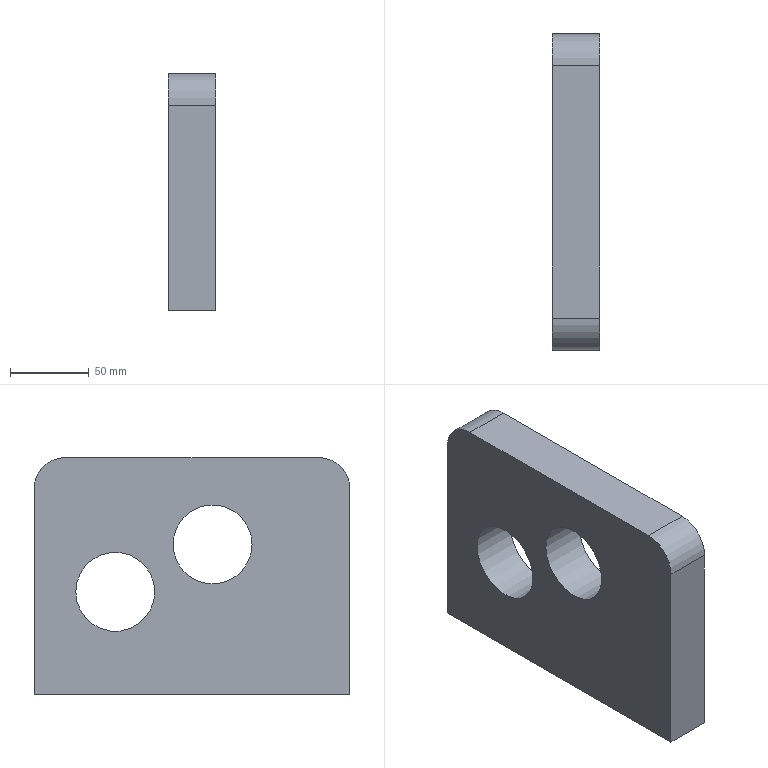Component | NX | TEMPLATE | 1 solid | 16 faces | box 30 x 200 x 150 mm | volume 766710 mm3 | plane 6 | cylinder 6 | cone 4 | commonest cylinder face diameters 50 x2 14 x2 40 x2
STEP:
#1=CARTESIAN_POINT('',(0.,0.,0.));
#2=DIRECTION('',(0.,0.,1.));
#3=DIRECTION('',(1.,0.,0.));
#4=AXIS2_PLACEMENT_3D('',#1,#2,#3);
#5=CARTESIAN_POINT('',(-275.,-100.,180.));
#6=VERTEX_POINT('',#5);
#7=CARTESIAN_POINT('',(-275.,-100.,50.));
#8=VERTEX_POINT('',#7);
#9=CARTESIAN_POINT('',(-275.,-100.,200.));
#10=DIRECTION('',(0.,-0.,-1.));
#11=VECTOR('',#10,1.);
#12=LINE('',#9,#11);
#13=CARTESIAN_POINT('',(-275.,-100.,200.));
#14=DIRECTION('',(0.,1.,-0.));
#15=DIRECTION('',(0.,-0.,-1.));
#16=AXIS2_PLACEMENT_3D('',#13,#14,#15);
#17=PLANE('',#16);
#18=CARTESIAN_POINT('',(0.,0.));
#19=DIRECTION('',(1.,0.));
#20=VECTOR('',#19,1.);
#21=LINE('',#18,#20);
#22=(GEOMETRIC_REPRESENTATION_CONTEXT(2)PARAMETRIC_REPRESENTATION_CONTEXT()REPRESENTATION_CONTEXT('',''));
#23=DEFINITIONAL_REPRESENTATION('',(#21),#22);
#24=PCURVE('',#17,#23);
#25=CARTESIAN_POINT('',(-275.,48.56,115.));
#26=DIRECTION('',(-1.,0.,0.));
#27=DIRECTION('',(0.,0.,1.));
#28=AXIS2_PLACEMENT_3D('',#25,#26,#27);
#29=PLANE('',#28);
#30=CARTESIAN_POINT('',(85.,-148.56));
#31=DIRECTION('',(-1.,-0.));
#32=VECTOR('',#31,1.);
#33=LINE('',#30,#32);
#34=(GEOMETRIC_REPRESENTATION_CONTEXT(2)PARAMETRIC_REPRESENTATION_CONTEXT()REPRESENTATION_CONTEXT('',''));
#35=DEFINITIONAL_REPRESENTATION('',(#33),#34);
#36=PCURVE('',#29,#35);
#37=SURFACE_CURVE('',#12,(#24,#36),.PCURVE_S1.);
#38=EDGE_CURVE('',#6,#8,#37,.T.);
#39=ORIENTED_EDGE('',*,*,#38,.F.);
#40=CARTESIAN_POINT('',(-305.,-100.,180.));
#41=VERTEX_POINT('',#40);
#42=CARTESIAN_POINT('',(-275.,-100.,180.));
#43=DIRECTION('',(-1.,0.,0.));
#44=VECTOR('',#43,1.);
#45=LINE('',#42,#44);
#46=CARTESIAN_POINT('',(20.,0.));
#47=DIRECTION('',(0.,1.));
#48=VECTOR('',#47,1.);
#49=LINE('',#46,#48);
#50=(GEOMETRIC_REPRESENTATION_CONTEXT(2)PARAMETRIC_REPRESENTATION_CONTEXT()REPRESENTATION_CONTEXT('',''));
#51=DEFINITIONAL_REPRESENTATION('',(#49),#50);
#52=PCURVE('',#17,#51);
#53=CARTESIAN_POINT('',(-275.,-80.,180.));
#54=DIRECTION('',(-1.,0.,0.));
#55=DIRECTION('',(0.,0.,1.));
#56=AXIS2_PLACEMENT_3D('',#53,#54,#55);
#57=CYLINDRICAL_SURFACE('',#56,20.);
#58=CARTESIAN_POINT('',(4.712,0.));
#59=DIRECTION('',(0.,1.));
#60=VECTOR('',#59,1.);
#61=LINE('',#58,#60);
#62=(GEOMETRIC_REPRESENTATION_CONTEXT(2)PARAMETRIC_REPRESENTATION_CONTEXT()REPRESENTATION_CONTEXT('',''));
#63=DEFINITIONAL_REPRESENTATION('',(#61),#62);
#64=PCURVE('',#57,#63);
#65=SURFACE_CURVE('',#45,(#52,#64),.PCURVE_S1.);
#66=EDGE_CURVE('',#6,#41,#65,.T.);
#67=ORIENTED_EDGE('',*,*,#66,.T.);
#68=CARTESIAN_POINT('',(-305.,-100.,50.));
#69=VERTEX_POINT('',#68);
#70=CARTESIAN_POINT('',(-305.,-100.,200.));
#71=DIRECTION('',(0.,-0.,-1.));
#72=VECTOR('',#71,1.);
#73=LINE('',#70,#72);
#74=CARTESIAN_POINT('',(0.,30.));
#75=DIRECTION('',(1.,0.));
#76=VECTOR('',#75,1.);
#77=LINE('',#74,#76);
#78=(GEOMETRIC_REPRESENTATION_CONTEXT(2)PARAMETRIC_REPRESENTATION_CONTEXT()REPRESENTATION_CONTEXT('',''));
#79=DEFINITIONAL_REPRESENTATION('',(#77),#78);
#80=PCURVE('',#17,#79);
#81=CARTESIAN_POINT('',(-305.,48.56,115.));
#82=DIRECTION('',(-1.,0.,0.));
#83=DIRECTION('',(0.,0.,1.));
#84=AXIS2_PLACEMENT_3D('',#81,#82,#83);
#85=PLANE('',#84);
#86=CARTESIAN_POINT('',(85.,-148.56));
#87=DIRECTION('',(-1.,-0.));
#88=VECTOR('',#87,1.);
#89=LINE('',#86,#88);
#90=(GEOMETRIC_REPRESENTATION_CONTEXT(2)PARAMETRIC_REPRESENTATION_CONTEXT()REPRESENTATION_CONTEXT('',''));
#91=DEFINITIONAL_REPRESENTATION('',(#89),#90);
#92=PCURVE('',#85,#91);
#93=SURFACE_CURVE('',#73,(#80,#92),.PCURVE_S1.);
#94=EDGE_CURVE('',#41,#69,#93,.T.);
#95=ORIENTED_EDGE('',*,*,#94,.T.);
#96=CARTESIAN_POINT('',(-275.,-100.,50.));
#97=DIRECTION('',(-1.,0.,0.));
#98=VECTOR('',#97,1.);
#99=LINE('',#96,#98);
#100=CARTESIAN_POINT('',(150.,0.));
#101=DIRECTION('',(0.,1.));
#102=VECTOR('',#101,1.);
#103=LINE('',#100,#102);
#104=(GEOMETRIC_REPRESENTATION_CONTEXT(2)PARAMETRIC_REPRESENTATION_CONTEXT()REPRESENTATION_CONTEXT('',''));
#105=DEFINITIONAL_REPRESENTATION('',(#103),#104);
#106=PCURVE('',#17,#105);
#107=CARTESIAN_POINT('',(-275.,-100.,50.));
#108=DIRECTION('',(0.,0.,1.));
#109=DIRECTION('',(1.,0.,0.));
#110=AXIS2_PLACEMENT_3D('',#107,#108,#109);
#111=PLANE('',#110);
#112=CARTESIAN_POINT('',(0.,0.));
#113=DIRECTION('',(-1.,0.));
#114=VECTOR('',#113,1.);
#115=LINE('',#112,#114);
#116=(GEOMETRIC_REPRESENTATION_CONTEXT(2)PARAMETRIC_REPRESENTATION_CONTEXT()REPRESENTATION_CONTEXT('',''));
#117=DEFINITIONAL_REPRESENTATION('',(#115),#116);
#118=PCURVE('',#111,#117);
#119=SURFACE_CURVE('',#99,(#106,#118),.PCURVE_S1.);
#120=EDGE_CURVE('',#8,#69,#119,.T.);
#121=ORIENTED_EDGE('',*,*,#120,.F.);
#122=EDGE_LOOP('',(#39,#67,#95,#121));
#123=FACE_BOUND('',#122,.T.);
#124=ADVANCED_FACE('',(#123),#17,.F.);
#125=CARTESIAN_POINT('',(-282.,50.,50.));
#126=VERTEX_POINT('',#125);
#127=CARTESIAN_POINT('',(-290.,50.,50.));
#128=DIRECTION('',(0.,0.,1.));
#129=DIRECTION('',(1.,0.,0.));
#130=AXIS2_PLACEMENT_3D('',#127,#128,#129);
#131=CIRCLE('',#130,8.);
#132=CARTESIAN_POINT('',(-15.,150.));
#133=DIRECTION('',(1.,0.));
#134=AXIS2_PLACEMENT_2D('',#132,#133);
#135=CIRCLE('',#134,8.);
#136=(GEOMETRIC_REPRESENTATION_CONTEXT(2)PARAMETRIC_REPRESENTATION_CONTEXT()REPRESENTATION_CONTEXT('',''));
#137=DEFINITIONAL_REPRESENTATION('',(#135),#136);
#138=PCURVE('',#111,#137);
#139=CARTESIAN_POINT('',(-290.,50.,50.));
#140=DIRECTION('',(0.,0.,-1.));
#141=DIRECTION('',(-1.,0.,0.));
#142=AXIS2_PLACEMENT_3D('',#139,#140,#141);
#143=CONICAL_SURFACE('',#142,8.,0.7854);
#144=CARTESIAN_POINT('',(9.425,0.));
#145=DIRECTION('',(-1.,0.));
#146=VECTOR('',#145,1.);
#147=LINE('',#144,#146);
#148=(GEOMETRIC_REPRESENTATION_CONTEXT(2)PARAMETRIC_REPRESENTATION_CONTEXT()REPRESENTATION_CONTEXT('',''));
#149=DEFINITIONAL_REPRESENTATION('',(#147),#148);
#150=PCURVE('',#143,#149);
#151=SURFACE_CURVE('',#131,(#138,#150),.PCURVE_S1.);
#152=EDGE_CURVE('',#126,#126,#151,.T.);
#153=ORIENTED_EDGE('',*,*,#152,.T.);
#154=EDGE_LOOP('',(#153));
#155=FACE_BOUND('',#154,.T.);
#156=CARTESIAN_POINT('',(-282.,-50.,50.));
#157=VERTEX_POINT('',#156);
#158=CARTESIAN_POINT('',(-290.,-50.,50.));
#159=DIRECTION('',(0.,0.,1.));
#160=DIRECTION('',(1.,0.,0.));
#161=AXIS2_PLACEMENT_3D('',#158,#159,#160);
#162=CIRCLE('',#161,8.);
#163=CARTESIAN_POINT('',(-15.,50.));
#164=DIRECTION('',(1.,0.));
#165=AXIS2_PLACEMENT_2D('',#163,#164);
#166=CIRCLE('',#165,8.);
#167=(GEOMETRIC_REPRESENTATION_CONTEXT(2)PARAMETRIC_REPRESENTATION_CONTEXT()REPRESENTATION_CONTEXT('',''));
#168=DEFINITIONAL_REPRESENTATION('',(#166),#167);
#169=PCURVE('',#111,#168);
#170=CARTESIAN_POINT('',(-290.,-50.,50.));
#171=DIRECTION('',(0.,0.,-1.));
#172=DIRECTION('',(-1.,0.,0.));
#173=AXIS2_PLACEMENT_3D('',#170,#171,#172);
#174=CONICAL_SURFACE('',#173,8.,0.7854);
#175=CARTESIAN_POINT('',(9.425,0.));
#176=DIRECTION('',(-1.,0.));
#177=VECTOR('',#176,1.);
#178=LINE('',#175,#177);
#179=(GEOMETRIC_REPRESENTATION_CONTEXT(2)PARAMETRIC_REPRESENTATION_CONTEXT()REPRESENTATION_CONTEXT('',''));
#180=DEFINITIONAL_REPRESENTATION('',(#178),#179);
#181=PCURVE('',#174,#180);
#182=SURFACE_CURVE('',#162,(#169,#181),.PCURVE_S1.);
#183=EDGE_CURVE('',#157,#157,#182,.T.);
#184=ORIENTED_EDGE('',*,*,#183,.T.);
#185=EDGE_LOOP('',(#184));
#186=FACE_BOUND('',#185,.T.);
#187=CARTESIAN_POINT('',(-305.,100.,50.));
#188=VERTEX_POINT('',#187);
#189=CARTESIAN_POINT('',(-305.,-100.,50.));
#190=DIRECTION('',(0.,1.,0.));
#191=VECTOR('',#190,1.);
#192=LINE('',#189,#191);
#193=CARTESIAN_POINT('',(-30.,0.));
#194=DIRECTION('',(0.,1.));
#195=VECTOR('',#194,1.);
#196=LINE('',#193,#195);
#197=(GEOMETRIC_REPRESENTATION_CONTEXT(2)PARAMETRIC_REPRESENTATION_CONTEXT()REPRESENTATION_CONTEXT('',''));
#198=DEFINITIONAL_REPRESENTATION('',(#196),#197);
#199=PCURVE('',#111,#198);
#200=CARTESIAN_POINT('',(-65.,-148.56));
#201=DIRECTION('',(0.,1.));
#202=VECTOR('',#201,1.);
#203=LINE('',#200,#202);
#204=(GEOMETRIC_REPRESENTATION_CONTEXT(2)PARAMETRIC_REPRESENTATION_CONTEXT()REPRESENTATION_CONTEXT('',''));
#205=DEFINITIONAL_REPRESENTATION('',(#203),#204);
#206=PCURVE('',#85,#205);
#207=SURFACE_CURVE('',#192,(#199,#206),.PCURVE_S1.);
#208=EDGE_CURVE('',#69,#188,#207,.T.);
#209=ORIENTED_EDGE('',*,*,#208,.T.);
#210=CARTESIAN_POINT('',(-275.,100.,50.));
#211=VERTEX_POINT('',#210);
#212=CARTESIAN_POINT('',(-275.,100.,50.));
#213=DIRECTION('',(-1.,0.,0.));
#214=VECTOR('',#213,1.);
#215=LINE('',#212,#214);
#216=CARTESIAN_POINT('',(0.,200.));
#217=DIRECTION('',(-1.,0.));
#218=VECTOR('',#217,1.);
#219=LINE('',#216,#218);
#220=(GEOMETRIC_REPRESENTATION_CONTEXT(2)PARAMETRIC_REPRESENTATION_CONTEXT()REPRESENTATION_CONTEXT('',''));
#221=DEFINITIONAL_REPRESENTATION('',(#219),#220);
#222=PCURVE('',#111,#221);
#223=CARTESIAN_POINT('',(-275.,100.,50.));
#224=DIRECTION('',(0.,-1.,-0.));
#225=DIRECTION('',(0.,-0.,1.));
#226=AXIS2_PLACEMENT_3D('',#223,#224,#225);
#227=PLANE('',#226);
#228=CARTESIAN_POINT('',(0.,0.));
#229=DIRECTION('',(0.,1.));
#230=VECTOR('',#229,1.);
#231=LINE('',#228,#230);
#232=(GEOMETRIC_REPRESENTATION_CONTEXT(2)PARAMETRIC_REPRESENTATION_CONTEXT()REPRESENTATION_CONTEXT('',''));
#233=DEFINITIONAL_REPRESENTATION('',(#231),#232);
#234=PCURVE('',#227,#233);
#235=SURFACE_CURVE('',#215,(#222,#234),.PCURVE_S1.);
#236=EDGE_CURVE('',#211,#188,#235,.T.);
#237=ORIENTED_EDGE('',*,*,#236,.F.);
#238=CARTESIAN_POINT('',(-275.,-100.,50.));
#239=DIRECTION('',(0.,1.,0.));
#240=VECTOR('',#239,1.);
#241=LINE('',#238,#240);
#242=CARTESIAN_POINT('',(0.,0.));
#243=DIRECTION('',(0.,1.));
#244=VECTOR('',#243,1.);
#245=LINE('',#242,#244);
#246=(GEOMETRIC_REPRESENTATION_CONTEXT(2)PARAMETRIC_REPRESENTATION_CONTEXT()REPRESENTATION_CONTEXT('',''));
#247=DEFINITIONAL_REPRESENTATION('',(#245),#246);
#248=PCURVE('',#111,#247);
#249=CARTESIAN_POINT('',(-65.,-148.56));
#250=DIRECTION('',(0.,1.));
#251=VECTOR('',#250,1.);
#252=LINE('',#249,#251);
#253=(GEOMETRIC_REPRESENTATION_CONTEXT(2)PARAMETRIC_REPRESENTATION_CONTEXT()REPRESENTATION_CONTEXT('',''));
#254=DEFINITIONAL_REPRESENTATION('',(#252),#253);
#255=PCURVE('',#29,#254);
#256=SURFACE_CURVE('',#241,(#248,#255),.PCURVE_S1.);
#257=EDGE_CURVE('',#8,#211,#256,.T.);
#258=ORIENTED_EDGE('',*,*,#257,.F.);
#259=ORIENTED_EDGE('',*,*,#120,.T.);
#260=EDGE_LOOP('',(#209,#237,#258,#259));
#261=FACE_BOUND('',#260,.T.);
#262=ADVANCED_FACE('',(#155,#186,#261),#111,.F.);
#263=CARTESIAN_POINT('',(-305.,100.,180.));
#264=VERTEX_POINT('',#263);
#265=CARTESIAN_POINT('',(-305.,100.,50.));
#266=DIRECTION('',(0.,-0.,1.));
#267=VECTOR('',#266,1.);
#268=LINE('',#265,#267);
#269=CARTESIAN_POINT('',(0.,30.));
#270=DIRECTION('',(1.,0.));
#271=VECTOR('',#270,1.);
#272=LINE('',#269,#271);
#273=(GEOMETRIC_REPRESENTATION_CONTEXT(2)PARAMETRIC_REPRESENTATION_CONTEXT()REPRESENTATION_CONTEXT('',''));
#274=DEFINITIONAL_REPRESENTATION('',(#272),#273);
#275=PCURVE('',#227,#274);
#276=CARTESIAN_POINT('',(-65.,51.44));
#277=DIRECTION('',(1.,-0.));
#278=VECTOR('',#277,1.);
#279=LINE('',#276,#278);
#280=(GEOMETRIC_REPRESENTATION_CONTEXT(2)PARAMETRIC_REPRESENTATION_CONTEXT()REPRESENTATION_CONTEXT('',''));
#281=DEFINITIONAL_REPRESENTATION('',(#279),#280);
#282=PCURVE('',#85,#281);
#283=SURFACE_CURVE('',#268,(#275,#282),.PCURVE_S1.);
#284=EDGE_CURVE('',#188,#264,#283,.T.);
#285=ORIENTED_EDGE('',*,*,#284,.T.);
#286=CARTESIAN_POINT('',(-275.,100.,180.));
#287=VERTEX_POINT('',#286);
#288=CARTESIAN_POINT('',(-275.,100.,180.));
#289=DIRECTION('',(1.,0.,0.));
#290=VECTOR('',#289,1.);
#291=LINE('',#288,#290);
#292=CARTESIAN_POINT('',(130.,0.));
#293=DIRECTION('',(0.,-1.));
#294=VECTOR('',#293,1.);
#295=LINE('',#292,#294);
#296=(GEOMETRIC_REPRESENTATION_CONTEXT(2)PARAMETRIC_REPRESENTATION_CONTEXT()REPRESENTATION_CONTEXT('',''));
#297=DEFINITIONAL_REPRESENTATION('',(#295),#296);
#298=PCURVE('',#227,#297);
#299=CARTESIAN_POINT('',(-275.,80.,180.));
#300=DIRECTION('',(-1.,0.,0.));
#301=DIRECTION('',(0.,0.,1.));
#302=AXIS2_PLACEMENT_3D('',#299,#300,#301);
#303=CYLINDRICAL_SURFACE('',#302,20.);
#304=CARTESIAN_POINT('',(1.571,0.));
#305=DIRECTION('',(0.,-1.));
#306=VECTOR('',#305,1.);
#307=LINE('',#304,#306);
#308=(GEOMETRIC_REPRESENTATION_CONTEXT(2)PARAMETRIC_REPRESENTATION_CONTEXT()REPRESENTATION_CONTEXT('',''));
#309=DEFINITIONAL_REPRESENTATION('',(#307),#308);
#310=PCURVE('',#303,#309);
#311=SURFACE_CURVE('',#291,(#298,#310),.PCURVE_S1.);
#312=EDGE_CURVE('',#264,#287,#311,.T.);
#313=ORIENTED_EDGE('',*,*,#312,.T.);
#314=CARTESIAN_POINT('',(-275.,100.,50.));
#315=DIRECTION('',(0.,-0.,1.));
#316=VECTOR('',#315,1.);
#317=LINE('',#314,#316);
#318=CARTESIAN_POINT('',(0.,0.));
#319=DIRECTION('',(1.,0.));
#320=VECTOR('',#319,1.);
#321=LINE('',#318,#320);
#322=(GEOMETRIC_REPRESENTATION_CONTEXT(2)PARAMETRIC_REPRESENTATION_CONTEXT()REPRESENTATION_CONTEXT('',''));
#323=DEFINITIONAL_REPRESENTATION('',(#321),#322);
#324=PCURVE('',#227,#323);
#325=CARTESIAN_POINT('',(-65.,51.44));
#326=DIRECTION('',(1.,-0.));
#327=VECTOR('',#326,1.);
#328=LINE('',#325,#327);
#329=(GEOMETRIC_REPRESENTATION_CONTEXT(2)PARAMETRIC_REPRESENTATION_CONTEXT()REPRESENTATION_CONTEXT('',''));
#330=DEFINITIONAL_REPRESENTATION('',(#328),#329);
#331=PCURVE('',#29,#330);
#332=SURFACE_CURVE('',#317,(#324,#331),.PCURVE_S1.);
#333=EDGE_CURVE('',#211,#287,#332,.T.);
#334=ORIENTED_EDGE('',*,*,#333,.F.);
#335=ORIENTED_EDGE('',*,*,#236,.T.);
#336=EDGE_LOOP('',(#285,#313,#334,#335));
#337=FACE_BOUND('',#336,.T.);
#338=ADVANCED_FACE('',(#337),#227,.F.);
#339=CARTESIAN_POINT('',(-275.,73.56,115.));
#340=VERTEX_POINT('',#339);
#341=CARTESIAN_POINT('',(-275.,48.56,115.));
#342=DIRECTION('',(-1.,0.,0.));
#343=DIRECTION('',(0.,1.,0.));
#344=AXIS2_PLACEMENT_3D('',#341,#342,#343);
#345=CIRCLE('',#344,25.);
#346=CARTESIAN_POINT('',(-275.,48.56,115.));
#347=DIRECTION('',(-1.,0.,0.));
#348=DIRECTION('',(0.,0.,1.));
#349=AXIS2_PLACEMENT_3D('',#346,#347,#348);
#350=CYLINDRICAL_SURFACE('',#349,25.);
#351=CARTESIAN_POINT('',(1.571,0.));
#352=DIRECTION('',(1.,0.));
#353=VECTOR('',#352,1.);
#354=LINE('',#351,#353);
#355=(GEOMETRIC_REPRESENTATION_CONTEXT(2)PARAMETRIC_REPRESENTATION_CONTEXT()REPRESENTATION_CONTEXT('',''));
#356=DEFINITIONAL_REPRESENTATION('',(#354),#355);
#357=PCURVE('',#350,#356);
#358=CARTESIAN_POINT('',(0.,0.));
#359=DIRECTION('',(0.,1.));
#360=AXIS2_PLACEMENT_2D('',#358,#359);
#361=CIRCLE('',#360,25.);
#362=(GEOMETRIC_REPRESENTATION_CONTEXT(2)PARAMETRIC_REPRESENTATION_CONTEXT()REPRESENTATION_CONTEXT('',''));
#363=DEFINITIONAL_REPRESENTATION('',(#361),#362);
#364=PCURVE('',#29,#363);
#365=SURFACE_CURVE('',#345,(#357,#364),.PCURVE_S1.);
#366=EDGE_CURVE('',#340,#340,#365,.T.);
#367=ORIENTED_EDGE('',*,*,#366,.T.);
#368=CARTESIAN_POINT('',(-305.,73.56,115.));
#369=VERTEX_POINT('',#368);
#370=CARTESIAN_POINT('',(-275.,73.56,115.));
#371=CARTESIAN_POINT('',(-305.,73.56,115.));
#372=B_SPLINE_CURVE_WITH_KNOTS('',1,(#370,#371),.UNSPECIFIED.,.F.,.F.,(2,2),(0.,30.),.PIECEWISE_BEZIER_KNOTS.);
#373=CARTESIAN_POINT('',(7.854,0.));
#374=DIRECTION('',(0.,1.));
#375=VECTOR('',#374,1.);
#376=LINE('',#373,#375);
#377=(GEOMETRIC_REPRESENTATION_CONTEXT(2)PARAMETRIC_REPRESENTATION_CONTEXT()REPRESENTATION_CONTEXT('',''));
#378=DEFINITIONAL_REPRESENTATION('',(#376),#377);
#379=PCURVE('',#350,#378);
#380=CARTESIAN_POINT('',(1.571,0.));
#381=DIRECTION('',(0.,1.));
#382=VECTOR('',#381,1.);
#383=LINE('',#380,#382);
#384=(GEOMETRIC_REPRESENTATION_CONTEXT(2)PARAMETRIC_REPRESENTATION_CONTEXT()REPRESENTATION_CONTEXT('',''));
#385=DEFINITIONAL_REPRESENTATION('',(#383),#384);
#386=PCURVE('',#350,#385);
#387=SEAM_CURVE('',#372,(#379,#386),.PCURVE_S1.);
#388=EDGE_CURVE('',#340,#369,#387,.T.);
#389=ORIENTED_EDGE('',*,*,#388,.T.);
#390=CARTESIAN_POINT('',(-305.,48.56,115.));
#391=DIRECTION('',(-1.,0.,0.));
#392=DIRECTION('',(0.,1.,0.));
#393=AXIS2_PLACEMENT_3D('',#390,#391,#392);
#394=CIRCLE('',#393,25.);
#395=CARTESIAN_POINT('',(1.571,30.));
#396=DIRECTION('',(1.,0.));
#397=VECTOR('',#396,1.);
#398=LINE('',#395,#397);
#399=(GEOMETRIC_REPRESENTATION_CONTEXT(2)PARAMETRIC_REPRESENTATION_CONTEXT()REPRESENTATION_CONTEXT('',''));
#400=DEFINITIONAL_REPRESENTATION('',(#398),#399);
#401=PCURVE('',#350,#400);
#402=CARTESIAN_POINT('',(0.,0.));
#403=DIRECTION('',(0.,1.));
#404=AXIS2_PLACEMENT_2D('',#402,#403);
#405=CIRCLE('',#404,25.);
#406=(GEOMETRIC_REPRESENTATION_CONTEXT(2)PARAMETRIC_REPRESENTATION_CONTEXT()REPRESENTATION_CONTEXT('',''));
#407=DEFINITIONAL_REPRESENTATION('',(#405),#406);
#408=PCURVE('',#85,#407);
#409=SURFACE_CURVE('',#394,(#401,#408),.PCURVE_S1.);
#410=EDGE_CURVE('',#369,#369,#409,.T.);
#411=ORIENTED_EDGE('',*,*,#410,.F.);
#412=ORIENTED_EDGE('',*,*,#388,.F.);
#413=EDGE_LOOP('',(#367,#389,#411,#412));
#414=FACE_BOUND('',#413,.F.);
#415=ADVANCED_FACE('',(#414),#350,.F.);
#416=CARTESIAN_POINT('',(-275.,80.,200.));
#417=VERTEX_POINT('',#416);
#418=CARTESIAN_POINT('',(-275.,-80.,200.));
#419=VERTEX_POINT('',#418);
#420=CARTESIAN_POINT('',(-275.,100.,200.));
#421=DIRECTION('',(0.,-1.,-0.));
#422=VECTOR('',#421,1.);
#423=LINE('',#420,#422);
#424=CARTESIAN_POINT('',(-275.,100.,200.));
#425=DIRECTION('',(0.,0.,-1.));
#426=DIRECTION('',(0.,-1.,-0.));
#427=AXIS2_PLACEMENT_3D('',#424,#425,#426);
#428=PLANE('',#427);
#429=CARTESIAN_POINT('',(0.,0.));
#430=DIRECTION('',(1.,0.));
#431=VECTOR('',#430,1.);
#432=LINE('',#429,#431);
#433=(GEOMETRIC_REPRESENTATION_CONTEXT(2)PARAMETRIC_REPRESENTATION_CONTEXT()REPRESENTATION_CONTEXT('',''));
#434=DEFINITIONAL_REPRESENTATION('',(#432),#433);
#435=PCURVE('',#428,#434);
#436=CARTESIAN_POINT('',(85.,51.44));
#437=DIRECTION('',(-0.,-1.));
#438=VECTOR('',#437,1.);
#439=LINE('',#436,#438);
#440=(GEOMETRIC_REPRESENTATION_CONTEXT(2)PARAMETRIC_REPRESENTATION_CONTEXT()REPRESENTATION_CONTEXT('',''));
#441=DEFINITIONAL_REPRESENTATION('',(#439),#440);
#442=PCURVE('',#29,#441);
#443=SURFACE_CURVE('',#423,(#435,#442),.PCURVE_S1.);
#444=EDGE_CURVE('',#417,#419,#443,.T.);
#445=ORIENTED_EDGE('',*,*,#444,.F.);
#446=CARTESIAN_POINT('',(-305.,80.,200.));
#447=VERTEX_POINT('',#446);
#448=CARTESIAN_POINT('',(-275.,80.,200.));
#449=DIRECTION('',(-1.,0.,0.));
#450=VECTOR('',#449,1.);
#451=LINE('',#448,#450);
#452=CARTESIAN_POINT('',(20.,0.));
#453=DIRECTION('',(0.,1.));
#454=VECTOR('',#453,1.);
#455=LINE('',#452,#454);
#456=(GEOMETRIC_REPRESENTATION_CONTEXT(2)PARAMETRIC_REPRESENTATION_CONTEXT()REPRESENTATION_CONTEXT('',''));
#457=DEFINITIONAL_REPRESENTATION('',(#455),#456);
#458=PCURVE('',#428,#457);
#459=CARTESIAN_POINT('',(0.,0.));
#460=DIRECTION('',(0.,1.));
#461=VECTOR('',#460,1.);
#462=LINE('',#459,#461);
#463=(GEOMETRIC_REPRESENTATION_CONTEXT(2)PARAMETRIC_REPRESENTATION_CONTEXT()REPRESENTATION_CONTEXT('',''));
#464=DEFINITIONAL_REPRESENTATION('',(#462),#463);
#465=PCURVE('',#303,#464);
#466=SURFACE_CURVE('',#451,(#458,#465),.PCURVE_S1.);
#467=EDGE_CURVE('',#417,#447,#466,.T.);
#468=ORIENTED_EDGE('',*,*,#467,.T.);
#469=CARTESIAN_POINT('',(-305.,-80.,200.));
#470=VERTEX_POINT('',#469);
#471=CARTESIAN_POINT('',(-305.,100.,200.));
#472=DIRECTION('',(0.,-1.,-0.));
#473=VECTOR('',#472,1.);
#474=LINE('',#471,#473);
#475=CARTESIAN_POINT('',(0.,30.));
#476=DIRECTION('',(1.,0.));
#477=VECTOR('',#476,1.);
#478=LINE('',#475,#477);
#479=(GEOMETRIC_REPRESENTATION_CONTEXT(2)PARAMETRIC_REPRESENTATION_CONTEXT()REPRESENTATION_CONTEXT('',''));
#480=DEFINITIONAL_REPRESENTATION('',(#478),#479);
#481=PCURVE('',#428,#480);
#482=CARTESIAN_POINT('',(85.,51.44));
#483=DIRECTION('',(-0.,-1.));
#484=VECTOR('',#483,1.);
#485=LINE('',#482,#484);
#486=(GEOMETRIC_REPRESENTATION_CONTEXT(2)PARAMETRIC_REPRESENTATION_CONTEXT()REPRESENTATION_CONTEXT('',''));
#487=DEFINITIONAL_REPRESENTATION('',(#485),#486);
#488=PCURVE('',#85,#487);
#489=SURFACE_CURVE('',#474,(#481,#488),.PCURVE_S1.);
#490=EDGE_CURVE('',#447,#470,#489,.T.);
#491=ORIENTED_EDGE('',*,*,#490,.T.);
#492=CARTESIAN_POINT('',(-275.,-80.,200.));
#493=DIRECTION('',(1.,0.,0.));
#494=VECTOR('',#493,1.);
#495=LINE('',#492,#494);
#496=CARTESIAN_POINT('',(180.,0.));
#497=DIRECTION('',(0.,-1.));
#498=VECTOR('',#497,1.);
#499=LINE('',#496,#498);
#500=(GEOMETRIC_REPRESENTATION_CONTEXT(2)PARAMETRIC_REPRESENTATION_CONTEXT()REPRESENTATION_CONTEXT('',''));
#501=DEFINITIONAL_REPRESENTATION('',(#499),#500);
#502=PCURVE('',#428,#501);
#503=CARTESIAN_POINT('',(6.283,0.));
#504=DIRECTION('',(0.,-1.));
#505=VECTOR('',#504,1.);
#506=LINE('',#503,#505);
#507=(GEOMETRIC_REPRESENTATION_CONTEXT(2)PARAMETRIC_REPRESENTATION_CONTEXT()REPRESENTATION_CONTEXT('',''));
#508=DEFINITIONAL_REPRESENTATION('',(#506),#507);
#509=PCURVE('',#57,#508);
#510=SURFACE_CURVE('',#495,(#502,#509),.PCURVE_S1.);
#511=EDGE_CURVE('',#470,#419,#510,.T.);
#512=ORIENTED_EDGE('',*,*,#511,.T.);
#513=EDGE_LOOP('',(#445,#468,#491,#512));
#514=FACE_BOUND('',#513,.T.);
#515=ADVANCED_FACE('',(#514),#428,.F.);
#516=CARTESIAN_POINT('',(-275.,12.,145.));
#517=VERTEX_POINT('',#516);
#518=CARTESIAN_POINT('',(-275.,-13.,145.));
#519=DIRECTION('',(-1.,0.,0.));
#520=DIRECTION('',(0.,1.,0.));
#521=AXIS2_PLACEMENT_3D('',#518,#519,#520);
#522=CIRCLE('',#521,25.);
#523=CARTESIAN_POINT('',(-275.,-13.,145.));
#524=DIRECTION('',(-1.,0.,0.));
#525=DIRECTION('',(0.,0.,1.));
#526=AXIS2_PLACEMENT_3D('',#523,#524,#525);
#527=CYLINDRICAL_SURFACE('',#526,25.);
#528=CARTESIAN_POINT('',(1.571,0.));
#529=DIRECTION('',(1.,0.));
#530=VECTOR('',#529,1.);
#531=LINE('',#528,#530);
#532=(GEOMETRIC_REPRESENTATION_CONTEXT(2)PARAMETRIC_REPRESENTATION_CONTEXT()REPRESENTATION_CONTEXT('',''));
#533=DEFINITIONAL_REPRESENTATION('',(#531),#532);
#534=PCURVE('',#527,#533);
#535=CARTESIAN_POINT('',(30.,-61.56));
#536=DIRECTION('',(0.,1.));
#537=AXIS2_PLACEMENT_2D('',#535,#536);
#538=CIRCLE('',#537,25.);
#539=(GEOMETRIC_REPRESENTATION_CONTEXT(2)PARAMETRIC_REPRESENTATION_CONTEXT()REPRESENTATION_CONTEXT('',''));
#540=DEFINITIONAL_REPRESENTATION('',(#538),#539);
#541=PCURVE('',#29,#540);
#542=SURFACE_CURVE('',#522,(#534,#541),.PCURVE_S1.);
#543=EDGE_CURVE('',#517,#517,#542,.T.);
#544=ORIENTED_EDGE('',*,*,#543,.T.);
#545=CARTESIAN_POINT('',(-305.,12.,145.));
#546=VERTEX_POINT('',#545);
#547=CARTESIAN_POINT('',(-275.,12.,145.));
#548=CARTESIAN_POINT('',(-305.,12.,145.));
#549=B_SPLINE_CURVE_WITH_KNOTS('',1,(#547,#548),.UNSPECIFIED.,.F.,.F.,(2,2),(0.,30.),.PIECEWISE_BEZIER_KNOTS.);
#550=CARTESIAN_POINT('',(7.854,0.));
#551=DIRECTION('',(0.,1.));
#552=VECTOR('',#551,1.);
#553=LINE('',#550,#552);
#554=(GEOMETRIC_REPRESENTATION_CONTEXT(2)PARAMETRIC_REPRESENTATION_CONTEXT()REPRESENTATION_CONTEXT('',''));
#555=DEFINITIONAL_REPRESENTATION('',(#553),#554);
#556=PCURVE('',#527,#555);
#557=CARTESIAN_POINT('',(1.571,0.));
#558=DIRECTION('',(0.,1.));
#559=VECTOR('',#558,1.);
#560=LINE('',#557,#559);
#561=(GEOMETRIC_REPRESENTATION_CONTEXT(2)PARAMETRIC_REPRESENTATION_CONTEXT()REPRESENTATION_CONTEXT('',''));
#562=DEFINITIONAL_REPRESENTATION('',(#560),#561);
#563=PCURVE('',#527,#562);
#564=SEAM_CURVE('',#549,(#556,#563),.PCURVE_S1.);
#565=EDGE_CURVE('',#517,#546,#564,.T.);
#566=ORIENTED_EDGE('',*,*,#565,.T.);
#567=CARTESIAN_POINT('',(-305.,-13.,145.));
#568=DIRECTION('',(-1.,0.,0.));
#569=DIRECTION('',(0.,1.,0.));
#570=AXIS2_PLACEMENT_3D('',#567,#568,#569);
#571=CIRCLE('',#570,25.);
#572=CARTESIAN_POINT('',(1.571,30.));
#573=DIRECTION('',(1.,0.));
#574=VECTOR('',#573,1.);
#575=LINE('',#572,#574);
#576=(GEOMETRIC_REPRESENTATION_CONTEXT(2)PARAMETRIC_REPRESENTATION_CONTEXT()REPRESENTATION_CONTEXT('',''));
#577=DEFINITIONAL_REPRESENTATION('',(#575),#576);
#578=PCURVE('',#527,#577);
#579=CARTESIAN_POINT('',(30.,-61.56));
#580=DIRECTION('',(0.,1.));
#581=AXIS2_PLACEMENT_2D('',#579,#580);
#582=CIRCLE('',#581,25.);
#583=(GEOMETRIC_REPRESENTATION_CONTEXT(2)PARAMETRIC_REPRESENTATION_CONTEXT()REPRESENTATION_CONTEXT('',''));
#584=DEFINITIONAL_REPRESENTATION('',(#582),#583);
#585=PCURVE('',#85,#584);
#586=SURFACE_CURVE('',#571,(#578,#585),.PCURVE_S1.);
#587=EDGE_CURVE('',#546,#546,#586,.T.);
#588=ORIENTED_EDGE('',*,*,#587,.F.);
#589=ORIENTED_EDGE('',*,*,#565,.F.);
#590=EDGE_LOOP('',(#544,#566,#588,#589));
#591=FACE_BOUND('',#590,.F.);
#592=ADVANCED_FACE('',(#591),#527,.F.);
#593=ORIENTED_EDGE('',*,*,#333,.T.);
#594=CARTESIAN_POINT('',(-275.,80.,180.));
#595=DIRECTION('',(1.,0.,0.));
#596=DIRECTION('',(0.,0.,1.));
#597=AXIS2_PLACEMENT_3D('',#594,#595,#596);
#598=CIRCLE('',#597,20.);
#599=CARTESIAN_POINT('',(85.,31.44));
#600=CARTESIAN_POINT('',(85.,-3.201));
#601=CARTESIAN_POINT('',(55.,14.119));
#602=CARTESIAN_POINT('',(25.,31.44));
#603=CARTESIAN_POINT('',(55.,48.761));
#604=CARTESIAN_POINT('',(85.,66.081));
#605=CARTESIAN_POINT('',(85.,31.44));
#606=(BOUNDED_CURVE()B_SPLINE_CURVE(2,(#599,#600,#601,#602,#603,#604,#605),.UNSPECIFIED.,.T.,.F.)B_SPLINE_CURVE_WITH_KNOTS((1,2,2,2,2,1),(-2.094,0.,2.094,4.189,6.283,8.378),.UNSPECIFIED.)CURVE()GEOMETRIC_REPRESENTATION_ITEM()RATIONAL_B_SPLINE_CURVE((1.,0.5,1.,0.5,1.,0.5,1.))REPRESENTATION_ITEM(''));
#607=(GEOMETRIC_REPRESENTATION_CONTEXT(2)PARAMETRIC_REPRESENTATION_CONTEXT()REPRESENTATION_CONTEXT('',''));
#608=DEFINITIONAL_REPRESENTATION('',(#606),#607);
#609=PCURVE('',#29,#608);
#610=CARTESIAN_POINT('',(6.283,0.));
#611=DIRECTION('',(-1.,0.));
#612=VECTOR('',#611,1.);
#613=LINE('',#610,#612);
#614=(GEOMETRIC_REPRESENTATION_CONTEXT(2)PARAMETRIC_REPRESENTATION_CONTEXT()REPRESENTATION_CONTEXT('',''));
#615=DEFINITIONAL_REPRESENTATION('',(#613),#614);
#616=PCURVE('',#303,#615);
#617=SURFACE_CURVE('',#598,(#609,#616),.PCURVE_S1.);
#618=EDGE_CURVE('',#287,#417,#617,.T.);
#619=ORIENTED_EDGE('',*,*,#618,.T.);
#620=ORIENTED_EDGE('',*,*,#444,.T.);
#621=CARTESIAN_POINT('',(-275.,-80.,180.));
#622=DIRECTION('',(1.,0.,0.));
#623=DIRECTION('',(0.,0.,1.));
#624=AXIS2_PLACEMENT_3D('',#621,#622,#623);
#625=CIRCLE('',#624,20.);
#626=CARTESIAN_POINT('',(85.,-128.56));
#627=CARTESIAN_POINT('',(85.,-163.201));
#628=CARTESIAN_POINT('',(55.,-145.881));
#629=CARTESIAN_POINT('',(25.,-128.56));
#630=CARTESIAN_POINT('',(55.,-111.239));
#631=CARTESIAN_POINT('',(85.,-93.919));
#632=CARTESIAN_POINT('',(85.,-128.56));
#633=(BOUNDED_CURVE()B_SPLINE_CURVE(2,(#626,#627,#628,#629,#630,#631,#632),.UNSPECIFIED.,.T.,.F.)B_SPLINE_CURVE_WITH_KNOTS((1,2,2,2,2,1),(-2.094,0.,2.094,4.189,6.283,8.378),.UNSPECIFIED.)CURVE()GEOMETRIC_REPRESENTATION_ITEM()RATIONAL_B_SPLINE_CURVE((1.,0.5,1.,0.5,1.,0.5,1.))REPRESENTATION_ITEM(''));
#634=(GEOMETRIC_REPRESENTATION_CONTEXT(2)PARAMETRIC_REPRESENTATION_CONTEXT()REPRESENTATION_CONTEXT('',''));
#635=DEFINITIONAL_REPRESENTATION('',(#633),#634);
#636=PCURVE('',#29,#635);
#637=CARTESIAN_POINT('',(6.283,0.));
#638=DIRECTION('',(-1.,0.));
#639=VECTOR('',#638,1.);
#640=LINE('',#637,#639);
#641=(GEOMETRIC_REPRESENTATION_CONTEXT(2)PARAMETRIC_REPRESENTATION_CONTEXT()REPRESENTATION_CONTEXT('',''));
#642=DEFINITIONAL_REPRESENTATION('',(#640),#641);
#643=PCURVE('',#57,#642);
#644=SURFACE_CURVE('',#625,(#636,#643),.PCURVE_S1.);
#645=EDGE_CURVE('',#419,#6,#644,.T.);
#646=ORIENTED_EDGE('',*,*,#645,.T.);
#647=ORIENTED_EDGE('',*,*,#38,.T.);
#648=ORIENTED_EDGE('',*,*,#257,.T.);
#649=EDGE_LOOP('',(#593,#619,#620,#646,#647,#648));
#650=FACE_BOUND('',#649,.T.);
#651=ORIENTED_EDGE('',*,*,#366,.T.);
#652=EDGE_LOOP('',(#651));
#653=FACE_BOUND('',#652,.T.);
#654=ORIENTED_EDGE('',*,*,#543,.T.);
#655=EDGE_LOOP('',(#654));
#656=FACE_BOUND('',#655,.T.);
#657=ADVANCED_FACE('',(#650,#653,#656),#29,.F.);
#658=ORIENTED_EDGE('',*,*,#490,.F.);
#659=CARTESIAN_POINT('',(-305.,80.,180.));
#660=DIRECTION('',(-1.,0.,0.));
#661=DIRECTION('',(0.,0.,1.));
#662=AXIS2_PLACEMENT_3D('',#659,#660,#661);
#663=CIRCLE('',#662,20.);
#664=CARTESIAN_POINT('',(65.,31.44));
#665=DIRECTION('',(1.,0.));
#666=AXIS2_PLACEMENT_2D('',#664,#665);
#667=CIRCLE('',#666,20.);
#668=(GEOMETRIC_REPRESENTATION_CONTEXT(2)PARAMETRIC_REPRESENTATION_CONTEXT()REPRESENTATION_CONTEXT('',''));
#669=DEFINITIONAL_REPRESENTATION('',(#667),#668);
#670=PCURVE('',#85,#669);
#671=CARTESIAN_POINT('',(0.,30.));
#672=DIRECTION('',(1.,0.));
#673=VECTOR('',#672,1.);
#674=LINE('',#671,#673);
#675=(GEOMETRIC_REPRESENTATION_CONTEXT(2)PARAMETRIC_REPRESENTATION_CONTEXT()REPRESENTATION_CONTEXT('',''));
#676=DEFINITIONAL_REPRESENTATION('',(#674),#675);
#677=PCURVE('',#303,#676);
#678=SURFACE_CURVE('',#663,(#670,#677),.PCURVE_S1.);
#679=EDGE_CURVE('',#447,#264,#678,.T.);
#680=ORIENTED_EDGE('',*,*,#679,.T.);
#681=ORIENTED_EDGE('',*,*,#284,.F.);
#682=ORIENTED_EDGE('',*,*,#208,.F.);
#683=ORIENTED_EDGE('',*,*,#94,.F.);
#684=CARTESIAN_POINT('',(-305.,-80.,180.));
#685=DIRECTION('',(-1.,0.,0.));
#686=DIRECTION('',(0.,0.,1.));
#687=AXIS2_PLACEMENT_3D('',#684,#685,#686);
#688=CIRCLE('',#687,20.);
#689=CARTESIAN_POINT('',(65.,-128.56));
#690=DIRECTION('',(1.,0.));
#691=AXIS2_PLACEMENT_2D('',#689,#690);
#692=CIRCLE('',#691,20.);
#693=(GEOMETRIC_REPRESENTATION_CONTEXT(2)PARAMETRIC_REPRESENTATION_CONTEXT()REPRESENTATION_CONTEXT('',''));
#694=DEFINITIONAL_REPRESENTATION('',(#692),#693);
#695=PCURVE('',#85,#694);
#696=CARTESIAN_POINT('',(0.,30.));
#697=DIRECTION('',(1.,0.));
#698=VECTOR('',#697,1.);
#699=LINE('',#696,#698);
#700=(GEOMETRIC_REPRESENTATION_CONTEXT(2)PARAMETRIC_REPRESENTATION_CONTEXT()REPRESENTATION_CONTEXT('',''));
#701=DEFINITIONAL_REPRESENTATION('',(#699),#700);
#702=PCURVE('',#57,#701);
#703=SURFACE_CURVE('',#688,(#695,#702),.PCURVE_S1.);
#704=EDGE_CURVE('',#41,#470,#703,.T.);
#705=ORIENTED_EDGE('',*,*,#704,.T.);
#706=EDGE_LOOP('',(#658,#680,#681,#682,#683,#705));
#707=FACE_BOUND('',#706,.T.);
#708=ORIENTED_EDGE('',*,*,#410,.F.);
#709=EDGE_LOOP('',(#708));
#710=FACE_BOUND('',#709,.T.);
#711=ORIENTED_EDGE('',*,*,#587,.F.);
#712=EDGE_LOOP('',(#711));
#713=FACE_BOUND('',#712,.T.);
#714=ADVANCED_FACE('',(#707,#710,#713),#85,.T.);
#715=CARTESIAN_POINT('',(-297.,-50.,82.));
#716=VERTEX_POINT('',#715);
#717=CARTESIAN_POINT('',(-283.,-50.,82.));
#718=VERTEX_POINT('',#717);
#719=CARTESIAN_POINT('',(-290.,-50.,82.));
#720=DIRECTION('',(0.,0.,-1.));
#721=DIRECTION('',(1.,0.,0.));
#722=AXIS2_PLACEMENT_3D('',#719,#720,#721);
#723=CIRCLE('',#722,7.);
#724=CARTESIAN_POINT('',(-290.,-50.,82.));
#725=DIRECTION('',(0.,0.,-1.));
#726=DIRECTION('',(-1.,0.,0.));
#727=AXIS2_PLACEMENT_3D('',#724,#725,#726);
#728=CONICAL_SURFACE('',#727,7.,1.03);
#729=CARTESIAN_POINT('',(-3.142,0.));
#730=DIRECTION('',(1.,0.));
#731=VECTOR('',#730,1.);
#732=LINE('',#729,#731);
#733=(GEOMETRIC_REPRESENTATION_CONTEXT(2)PARAMETRIC_REPRESENTATION_CONTEXT()REPRESENTATION_CONTEXT('',''));
#734=DEFINITIONAL_REPRESENTATION('',(#732),#733);
#735=PCURVE('',#728,#734);
#736=CARTESIAN_POINT('',(-290.,-50.,50.));
#737=DIRECTION('',(0.,0.,1.));
#738=DIRECTION('',(1.,0.,0.));
#739=AXIS2_PLACEMENT_3D('',#736,#737,#738);
#740=CYLINDRICAL_SURFACE('',#739,7.);
#741=CARTESIAN_POINT('',(6.283,32.));
#742=DIRECTION('',(-1.,0.));
#743=VECTOR('',#742,1.);
#744=LINE('',#741,#743);
#745=(GEOMETRIC_REPRESENTATION_CONTEXT(2)PARAMETRIC_REPRESENTATION_CONTEXT()REPRESENTATION_CONTEXT('',''));
#746=DEFINITIONAL_REPRESENTATION('',(#744),#745);
#747=PCURVE('',#740,#746);
#748=SURFACE_CURVE('',#723,(#735,#747),.PCURVE_S1.);
#749=EDGE_CURVE('',#716,#718,#748,.T.);
#750=ORIENTED_EDGE('',*,*,#749,.F.);
#751=CARTESIAN_POINT('',(-290.,-50.,86.206));
#752=VERTEX_POINT('',#751);
#753=CARTESIAN_POINT('',(-290.,-50.,86.206));
#754=CARTESIAN_POINT('',(-297.,-50.,82.));
#755=B_SPLINE_CURVE_WITH_KNOTS('',1,(#753,#754),.UNSPECIFIED.,.F.,.F.,(2,2),(-8.166,0.),.PIECEWISE_BEZIER_KNOTS.);
#756=CARTESIAN_POINT('',(0.,0.));
#757=DIRECTION('',(0.,1.));
#758=VECTOR('',#757,1.);
#759=LINE('',#756,#758);
#760=(GEOMETRIC_REPRESENTATION_CONTEXT(2)PARAMETRIC_REPRESENTATION_CONTEXT()REPRESENTATION_CONTEXT('',''));
#761=DEFINITIONAL_REPRESENTATION('',(#759),#760);
#762=PCURVE('',#728,#761);
#763=CARTESIAN_POINT('',(6.283,0.));
#764=DIRECTION('',(0.,1.));
#765=VECTOR('',#764,1.);
#766=LINE('',#763,#765);
#767=(GEOMETRIC_REPRESENTATION_CONTEXT(2)PARAMETRIC_REPRESENTATION_CONTEXT()REPRESENTATION_CONTEXT('',''));
#768=DEFINITIONAL_REPRESENTATION('',(#766),#767);
#769=PCURVE('',#728,#768);
#770=SEAM_CURVE('',#755,(#762,#769),.PCURVE_S1.);
#771=EDGE_CURVE('',#752,#716,#770,.T.);
#772=ORIENTED_EDGE('',*,*,#771,.F.);
#773=ORIENTED_EDGE('',*,*,#771,.T.);
#774=CARTESIAN_POINT('',(-290.,-50.,82.));
#775=DIRECTION('',(0.,0.,-1.));
#776=DIRECTION('',(1.,0.,0.));
#777=AXIS2_PLACEMENT_3D('',#774,#775,#776);
#778=CIRCLE('',#777,7.);
#779=CARTESIAN_POINT('',(3.142,0.));
#780=DIRECTION('',(1.,0.));
#781=VECTOR('',#780,1.);
#782=LINE('',#779,#781);
#783=(GEOMETRIC_REPRESENTATION_CONTEXT(2)PARAMETRIC_REPRESENTATION_CONTEXT()REPRESENTATION_CONTEXT('',''));
#784=DEFINITIONAL_REPRESENTATION('',(#782),#783);
#785=PCURVE('',#728,#784);
#786=CARTESIAN_POINT('',(6.283,32.));
#787=DIRECTION('',(-1.,0.));
#788=VECTOR('',#787,1.);
#789=LINE('',#786,#788);
#790=(GEOMETRIC_REPRESENTATION_CONTEXT(2)PARAMETRIC_REPRESENTATION_CONTEXT()REPRESENTATION_CONTEXT('',''));
#791=DEFINITIONAL_REPRESENTATION('',(#789),#790);
#792=PCURVE('',#740,#791);
#793=SURFACE_CURVE('',#778,(#785,#792),.PCURVE_S1.);
#794=EDGE_CURVE('',#718,#716,#793,.T.);
#795=ORIENTED_EDGE('',*,*,#794,.F.);
#796=EDGE_LOOP('',(#750,#772,#773,#795));
#797=FACE_BOUND('',#796,.F.);
#798=ADVANCED_FACE('',(#797),#728,.F.);
#799=CARTESIAN_POINT('',(-283.,-50.,51.));
#800=VERTEX_POINT('',#799);
#801=CARTESIAN_POINT('',(-290.,-50.,51.));
#802=DIRECTION('',(0.,0.,-1.));
#803=DIRECTION('',(1.,0.,0.));
#804=AXIS2_PLACEMENT_3D('',#801,#802,#803);
#805=CIRCLE('',#804,7.);
#806=CARTESIAN_POINT('',(6.283,1.));
#807=DIRECTION('',(-1.,0.));
#808=VECTOR('',#807,1.);
#809=LINE('',#806,#808);
#810=(GEOMETRIC_REPRESENTATION_CONTEXT(2)PARAMETRIC_REPRESENTATION_CONTEXT()REPRESENTATION_CONTEXT('',''));
#811=DEFINITIONAL_REPRESENTATION('',(#809),#810);
#812=PCURVE('',#740,#811);
#813=CARTESIAN_POINT('',(3.142,-1.));
#814=DIRECTION('',(1.,0.));
#815=VECTOR('',#814,1.);
#816=LINE('',#813,#815);
#817=(GEOMETRIC_REPRESENTATION_CONTEXT(2)PARAMETRIC_REPRESENTATION_CONTEXT()REPRESENTATION_CONTEXT('',''));
#818=DEFINITIONAL_REPRESENTATION('',(#816),#817);
#819=PCURVE('',#174,#818);
#820=SURFACE_CURVE('',#805,(#812,#819),.PCURVE_S1.);
#821=EDGE_CURVE('',#800,#800,#820,.T.);
#822=ORIENTED_EDGE('',*,*,#821,.F.);
#823=CARTESIAN_POINT('',(-283.,-50.,51.));
#824=CARTESIAN_POINT('',(-283.,-50.,82.));
#825=B_SPLINE_CURVE_WITH_KNOTS('',1,(#823,#824),.UNSPECIFIED.,.F.,.F.,(2,2),(1.,32.),.PIECEWISE_BEZIER_KNOTS.);
#826=CARTESIAN_POINT('',(6.283,0.));
#827=DIRECTION('',(0.,1.));
#828=VECTOR('',#827,1.);
#829=LINE('',#826,#828);
#830=(GEOMETRIC_REPRESENTATION_CONTEXT(2)PARAMETRIC_REPRESENTATION_CONTEXT()REPRESENTATION_CONTEXT('',''));
#831=DEFINITIONAL_REPRESENTATION('',(#829),#830);
#832=PCURVE('',#740,#831);
#833=CARTESIAN_POINT('',(0.,0.));
#834=DIRECTION('',(0.,1.));
#835=VECTOR('',#834,1.);
#836=LINE('',#833,#835);
#837=(GEOMETRIC_REPRESENTATION_CONTEXT(2)PARAMETRIC_REPRESENTATION_CONTEXT()REPRESENTATION_CONTEXT('',''));
#838=DEFINITIONAL_REPRESENTATION('',(#836),#837);
#839=PCURVE('',#740,#838);
#840=SEAM_CURVE('',#825,(#832,#839),.PCURVE_S1.);
#841=EDGE_CURVE('',#800,#718,#840,.T.);
#842=ORIENTED_EDGE('',*,*,#841,.T.);
#843=ORIENTED_EDGE('',*,*,#794,.T.);
#844=ORIENTED_EDGE('',*,*,#749,.T.);
#845=ORIENTED_EDGE('',*,*,#841,.F.);
#846=EDGE_LOOP('',(#822,#842,#843,#844,#845));
#847=FACE_BOUND('',#846,.F.);
#848=ADVANCED_FACE('',(#847),#740,.F.);
#849=ORIENTED_EDGE('',*,*,#821,.T.);
#850=CARTESIAN_POINT('',(-283.,-50.,51.));
#851=CARTESIAN_POINT('',(-282.,-50.,50.));
#852=B_SPLINE_CURVE_WITH_KNOTS('',1,(#850,#851),.UNSPECIFIED.,.F.,.F.,(2,2),(-1.414,0.),.PIECEWISE_BEZIER_KNOTS.);
#853=CARTESIAN_POINT('',(9.425,0.));
#854=DIRECTION('',(0.,1.));
#855=VECTOR('',#854,1.);
#856=LINE('',#853,#855);
#857=(GEOMETRIC_REPRESENTATION_CONTEXT(2)PARAMETRIC_REPRESENTATION_CONTEXT()REPRESENTATION_CONTEXT('',''));
#858=DEFINITIONAL_REPRESENTATION('',(#856),#857);
#859=PCURVE('',#174,#858);
#860=CARTESIAN_POINT('',(3.142,0.));
#861=DIRECTION('',(0.,1.));
#862=VECTOR('',#861,1.);
#863=LINE('',#860,#862);
#864=(GEOMETRIC_REPRESENTATION_CONTEXT(2)PARAMETRIC_REPRESENTATION_CONTEXT()REPRESENTATION_CONTEXT('',''));
#865=DEFINITIONAL_REPRESENTATION('',(#863),#864);
#866=PCURVE('',#174,#865);
#867=SEAM_CURVE('',#852,(#859,#866),.PCURVE_S1.);
#868=EDGE_CURVE('',#800,#157,#867,.T.);
#869=ORIENTED_EDGE('',*,*,#868,.T.);
#870=ORIENTED_EDGE('',*,*,#183,.T.);
#871=ORIENTED_EDGE('',*,*,#868,.F.);
#872=EDGE_LOOP('',(#849,#869,#870,#871));
#873=FACE_BOUND('',#872,.F.);
#874=ADVANCED_FACE('',(#873),#174,.F.);
#875=CARTESIAN_POINT('',(-297.,50.,82.));
#876=VERTEX_POINT('',#875);
#877=CARTESIAN_POINT('',(-283.,50.,82.));
#878=VERTEX_POINT('',#877);
#879=CARTESIAN_POINT('',(-290.,50.,82.));
#880=DIRECTION('',(0.,0.,-1.));
#881=DIRECTION('',(1.,0.,0.));
#882=AXIS2_PLACEMENT_3D('',#879,#880,#881);
#883=CIRCLE('',#882,7.);
#884=CARTESIAN_POINT('',(-290.,50.,82.));
#885=DIRECTION('',(0.,0.,-1.));
#886=DIRECTION('',(-1.,0.,0.));
#887=AXIS2_PLACEMENT_3D('',#884,#885,#886);
#888=CONICAL_SURFACE('',#887,7.,1.03);
#889=CARTESIAN_POINT('',(-3.142,0.));
#890=DIRECTION('',(1.,0.));
#891=VECTOR('',#890,1.);
#892=LINE('',#889,#891);
#893=(GEOMETRIC_REPRESENTATION_CONTEXT(2)PARAMETRIC_REPRESENTATION_CONTEXT()REPRESENTATION_CONTEXT('',''));
#894=DEFINITIONAL_REPRESENTATION('',(#892),#893);
#895=PCURVE('',#888,#894);
#896=CARTESIAN_POINT('',(-290.,50.,50.));
#897=DIRECTION('',(0.,0.,1.));
#898=DIRECTION('',(1.,0.,0.));
#899=AXIS2_PLACEMENT_3D('',#896,#897,#898);
#900=CYLINDRICAL_SURFACE('',#899,7.);
#901=CARTESIAN_POINT('',(6.283,32.));
#902=DIRECTION('',(-1.,0.));
#903=VECTOR('',#902,1.);
#904=LINE('',#901,#903);
#905=(GEOMETRIC_REPRESENTATION_CONTEXT(2)PARAMETRIC_REPRESENTATION_CONTEXT()REPRESENTATION_CONTEXT('',''));
#906=DEFINITIONAL_REPRESENTATION('',(#904),#905);
#907=PCURVE('',#900,#906);
#908=SURFACE_CURVE('',#883,(#895,#907),.PCURVE_S1.);
#909=EDGE_CURVE('',#876,#878,#908,.T.);
#910=ORIENTED_EDGE('',*,*,#909,.F.);
#911=CARTESIAN_POINT('',(-290.,50.,86.206));
#912=VERTEX_POINT('',#911);
#913=CARTESIAN_POINT('',(-290.,50.,86.206));
#914=CARTESIAN_POINT('',(-297.,50.,82.));
#915=B_SPLINE_CURVE_WITH_KNOTS('',1,(#913,#914),.UNSPECIFIED.,.F.,.F.,(2,2),(-8.166,0.),.PIECEWISE_BEZIER_KNOTS.);
#916=CARTESIAN_POINT('',(0.,0.));
#917=DIRECTION('',(0.,1.));
#918=VECTOR('',#917,1.);
#919=LINE('',#916,#918);
#920=(GEOMETRIC_REPRESENTATION_CONTEXT(2)PARAMETRIC_REPRESENTATION_CONTEXT()REPRESENTATION_CONTEXT('',''));
#921=DEFINITIONAL_REPRESENTATION('',(#919),#920);
#922=PCURVE('',#888,#921);
#923=CARTESIAN_POINT('',(6.283,0.));
#924=DIRECTION('',(0.,1.));
#925=VECTOR('',#924,1.);
#926=LINE('',#923,#925);
#927=(GEOMETRIC_REPRESENTATION_CONTEXT(2)PARAMETRIC_REPRESENTATION_CONTEXT()REPRESENTATION_CONTEXT('',''));
#928=DEFINITIONAL_REPRESENTATION('',(#926),#927);
#929=PCURVE('',#888,#928);
#930=SEAM_CURVE('',#915,(#922,#929),.PCURVE_S1.);
#931=EDGE_CURVE('',#912,#876,#930,.T.);
#932=ORIENTED_EDGE('',*,*,#931,.F.);
#933=ORIENTED_EDGE('',*,*,#931,.T.);
#934=CARTESIAN_POINT('',(-290.,50.,82.));
#935=DIRECTION('',(0.,0.,-1.));
#936=DIRECTION('',(1.,0.,0.));
#937=AXIS2_PLACEMENT_3D('',#934,#935,#936);
#938=CIRCLE('',#937,7.);
#939=CARTESIAN_POINT('',(3.142,0.));
#940=DIRECTION('',(1.,0.));
#941=VECTOR('',#940,1.);
#942=LINE('',#939,#941);
#943=(GEOMETRIC_REPRESENTATION_CONTEXT(2)PARAMETRIC_REPRESENTATION_CONTEXT()REPRESENTATION_CONTEXT('',''));
#944=DEFINITIONAL_REPRESENTATION('',(#942),#943);
#945=PCURVE('',#888,#944);
#946=CARTESIAN_POINT('',(6.283,32.));
#947=DIRECTION('',(-1.,0.));
#948=VECTOR('',#947,1.);
#949=LINE('',#946,#948);
#950=(GEOMETRIC_REPRESENTATION_CONTEXT(2)PARAMETRIC_REPRESENTATION_CONTEXT()REPRESENTATION_CONTEXT('',''));
#951=DEFINITIONAL_REPRESENTATION('',(#949),#950);
#952=PCURVE('',#900,#951);
#953=SURFACE_CURVE('',#938,(#945,#952),.PCURVE_S1.);
#954=EDGE_CURVE('',#878,#876,#953,.T.);
#955=ORIENTED_EDGE('',*,*,#954,.F.);
#956=EDGE_LOOP('',(#910,#932,#933,#955));
#957=FACE_BOUND('',#956,.F.);
#958=ADVANCED_FACE('',(#957),#888,.F.);
#959=CARTESIAN_POINT('',(-283.,50.,51.));
#960=VERTEX_POINT('',#959);
#961=CARTESIAN_POINT('',(-290.,50.,51.));
#962=DIRECTION('',(0.,0.,-1.));
#963=DIRECTION('',(1.,0.,0.));
#964=AXIS2_PLACEMENT_3D('',#961,#962,#963);
#965=CIRCLE('',#964,7.);
#966=CARTESIAN_POINT('',(6.283,1.));
#967=DIRECTION('',(-1.,0.));
#968=VECTOR('',#967,1.);
#969=LINE('',#966,#968);
#970=(GEOMETRIC_REPRESENTATION_CONTEXT(2)PARAMETRIC_REPRESENTATION_CONTEXT()REPRESENTATION_CONTEXT('',''));
#971=DEFINITIONAL_REPRESENTATION('',(#969),#970);
#972=PCURVE('',#900,#971);
#973=CARTESIAN_POINT('',(3.142,-1.));
#974=DIRECTION('',(1.,0.));
#975=VECTOR('',#974,1.);
#976=LINE('',#973,#975);
#977=(GEOMETRIC_REPRESENTATION_CONTEXT(2)PARAMETRIC_REPRESENTATION_CONTEXT()REPRESENTATION_CONTEXT('',''));
#978=DEFINITIONAL_REPRESENTATION('',(#976),#977);
#979=PCURVE('',#143,#978);
#980=SURFACE_CURVE('',#965,(#972,#979),.PCURVE_S1.);
#981=EDGE_CURVE('',#960,#960,#980,.T.);
#982=ORIENTED_EDGE('',*,*,#981,.F.);
#983=CARTESIAN_POINT('',(-283.,50.,51.));
#984=CARTESIAN_POINT('',(-283.,50.,82.));
#985=B_SPLINE_CURVE_WITH_KNOTS('',1,(#983,#984),.UNSPECIFIED.,.F.,.F.,(2,2),(1.,32.),.PIECEWISE_BEZIER_KNOTS.);
#986=CARTESIAN_POINT('',(6.283,0.));
#987=DIRECTION('',(0.,1.));
#988=VECTOR('',#987,1.);
#989=LINE('',#986,#988);
#990=(GEOMETRIC_REPRESENTATION_CONTEXT(2)PARAMETRIC_REPRESENTATION_CONTEXT()REPRESENTATION_CONTEXT('',''));
#991=DEFINITIONAL_REPRESENTATION('',(#989),#990);
#992=PCURVE('',#900,#991);
#993=CARTESIAN_POINT('',(0.,0.));
#994=DIRECTION('',(0.,1.));
#995=VECTOR('',#994,1.);
#996=LINE('',#993,#995);
#997=(GEOMETRIC_REPRESENTATION_CONTEXT(2)PARAMETRIC_REPRESENTATION_CONTEXT()REPRESENTATION_CONTEXT('',''));
#998=DEFINITIONAL_REPRESENTATION('',(#996),#997);
#999=PCURVE('',#900,#998);
#1000=SEAM_CURVE('',#985,(#992,#999),.PCURVE_S1.);
#1001=EDGE_CURVE('',#960,#878,#1000,.T.);
#1002=ORIENTED_EDGE('',*,*,#1001,.T.);
#1003=ORIENTED_EDGE('',*,*,#954,.T.);
#1004=ORIENTED_EDGE('',*,*,#909,.T.);
#1005=ORIENTED_EDGE('',*,*,#1001,.F.);
#1006=EDGE_LOOP('',(#982,#1002,#1003,#1004,#1005));
#1007=FACE_BOUND('',#1006,.F.);
#1008=ADVANCED_FACE('',(#1007),#900,.F.);
#1009=ORIENTED_EDGE('',*,*,#981,.T.);
#1010=CARTESIAN_POINT('',(-283.,50.,51.));
#1011=CARTESIAN_POINT('',(-282.,50.,50.));
#1012=B_SPLINE_CURVE_WITH_KNOTS('',1,(#1010,#1011),.UNSPECIFIED.,.F.,.F.,(2,2),(-1.414,0.),.PIECEWISE_BEZIER_KNOTS.);
#1013=CARTESIAN_POINT('',(9.425,0.));
#1014=DIRECTION('',(0.,1.));
#1015=VECTOR('',#1014,1.);
#1016=LINE('',#1013,#1015);
#1017=(GEOMETRIC_REPRESENTATION_CONTEXT(2)PARAMETRIC_REPRESENTATION_CONTEXT()REPRESENTATION_CONTEXT('',''));
#1018=DEFINITIONAL_REPRESENTATION('',(#1016),#1017);
#1019=PCURVE('',#143,#1018);
#1020=CARTESIAN_POINT('',(3.142,0.));
#1021=DIRECTION('',(0.,1.));
#1022=VECTOR('',#1021,1.);
#1023=LINE('',#1020,#1022);
#1024=(GEOMETRIC_REPRESENTATION_CONTEXT(2)PARAMETRIC_REPRESENTATION_CONTEXT()REPRESENTATION_CONTEXT('',''));
#1025=DEFINITIONAL_REPRESENTATION('',(#1023),#1024);
#1026=PCURVE('',#143,#1025);
#1027=SEAM_CURVE('',#1012,(#1019,#1026),.PCURVE_S1.);
#1028=EDGE_CURVE('',#960,#126,#1027,.T.);
#1029=ORIENTED_EDGE('',*,*,#1028,.T.);
#1030=ORIENTED_EDGE('',*,*,#152,.T.);
#1031=ORIENTED_EDGE('',*,*,#1028,.F.);
#1032=EDGE_LOOP('',(#1009,#1029,#1030,#1031));
#1033=FACE_BOUND('',#1032,.F.);
#1034=ADVANCED_FACE('',(#1033),#143,.F.);
#1035=ORIENTED_EDGE('',*,*,#618,.F.);
#1036=ORIENTED_EDGE('',*,*,#312,.F.);
#1037=ORIENTED_EDGE('',*,*,#679,.F.);
#1038=ORIENTED_EDGE('',*,*,#467,.F.);
#1039=EDGE_LOOP('',(#1035,#1036,#1037,#1038));
#1040=FACE_BOUND('',#1039,.T.);
#1041=ADVANCED_FACE('',(#1040),#303,.T.);
#1042=ORIENTED_EDGE('',*,*,#645,.F.);
#1043=ORIENTED_EDGE('',*,*,#511,.F.);
#1044=ORIENTED_EDGE('',*,*,#704,.F.);
#1045=ORIENTED_EDGE('',*,*,#66,.F.);
#1046=EDGE_LOOP('',(#1042,#1043,#1044,#1045));
#1047=FACE_BOUND('',#1046,.T.);
#1048=ADVANCED_FACE('',(#1047),#57,.T.);
#1049=CLOSED_SHELL('',(#124,#262,#338,#415,#515,#592,#657,#714,#798,#848,#874,#958,#1008,#1034,#1041,#1048));
#1050=MANIFOLD_SOLID_BREP('',#1049);
#1051=(LENGTH_UNIT()NAMED_UNIT(*)SI_UNIT(.MILLI.,.METRE.));
#1052=UNCERTAINTY_MEASURE_WITH_UNIT(LENGTH_MEASURE(0.000005),#1051,'','');
#1053=(NAMED_UNIT(*)PLANE_ANGLE_UNIT()SI_UNIT($,.RADIAN.));
#1054=(NAMED_UNIT(*)SI_UNIT($,.STERADIAN.)SOLID_ANGLE_UNIT());
#1055=(GEOMETRIC_REPRESENTATION_CONTEXT(3)GLOBAL_UNCERTAINTY_ASSIGNED_CONTEXT((#1052))GLOBAL_UNIT_ASSIGNED_CONTEXT((#1051,#1053,#1054))REPRESENTATION_CONTEXT('',''));
#1056=ADVANCED_BREP_SHAPE_REPRESENTATION('',(#4,#1050),#1055);